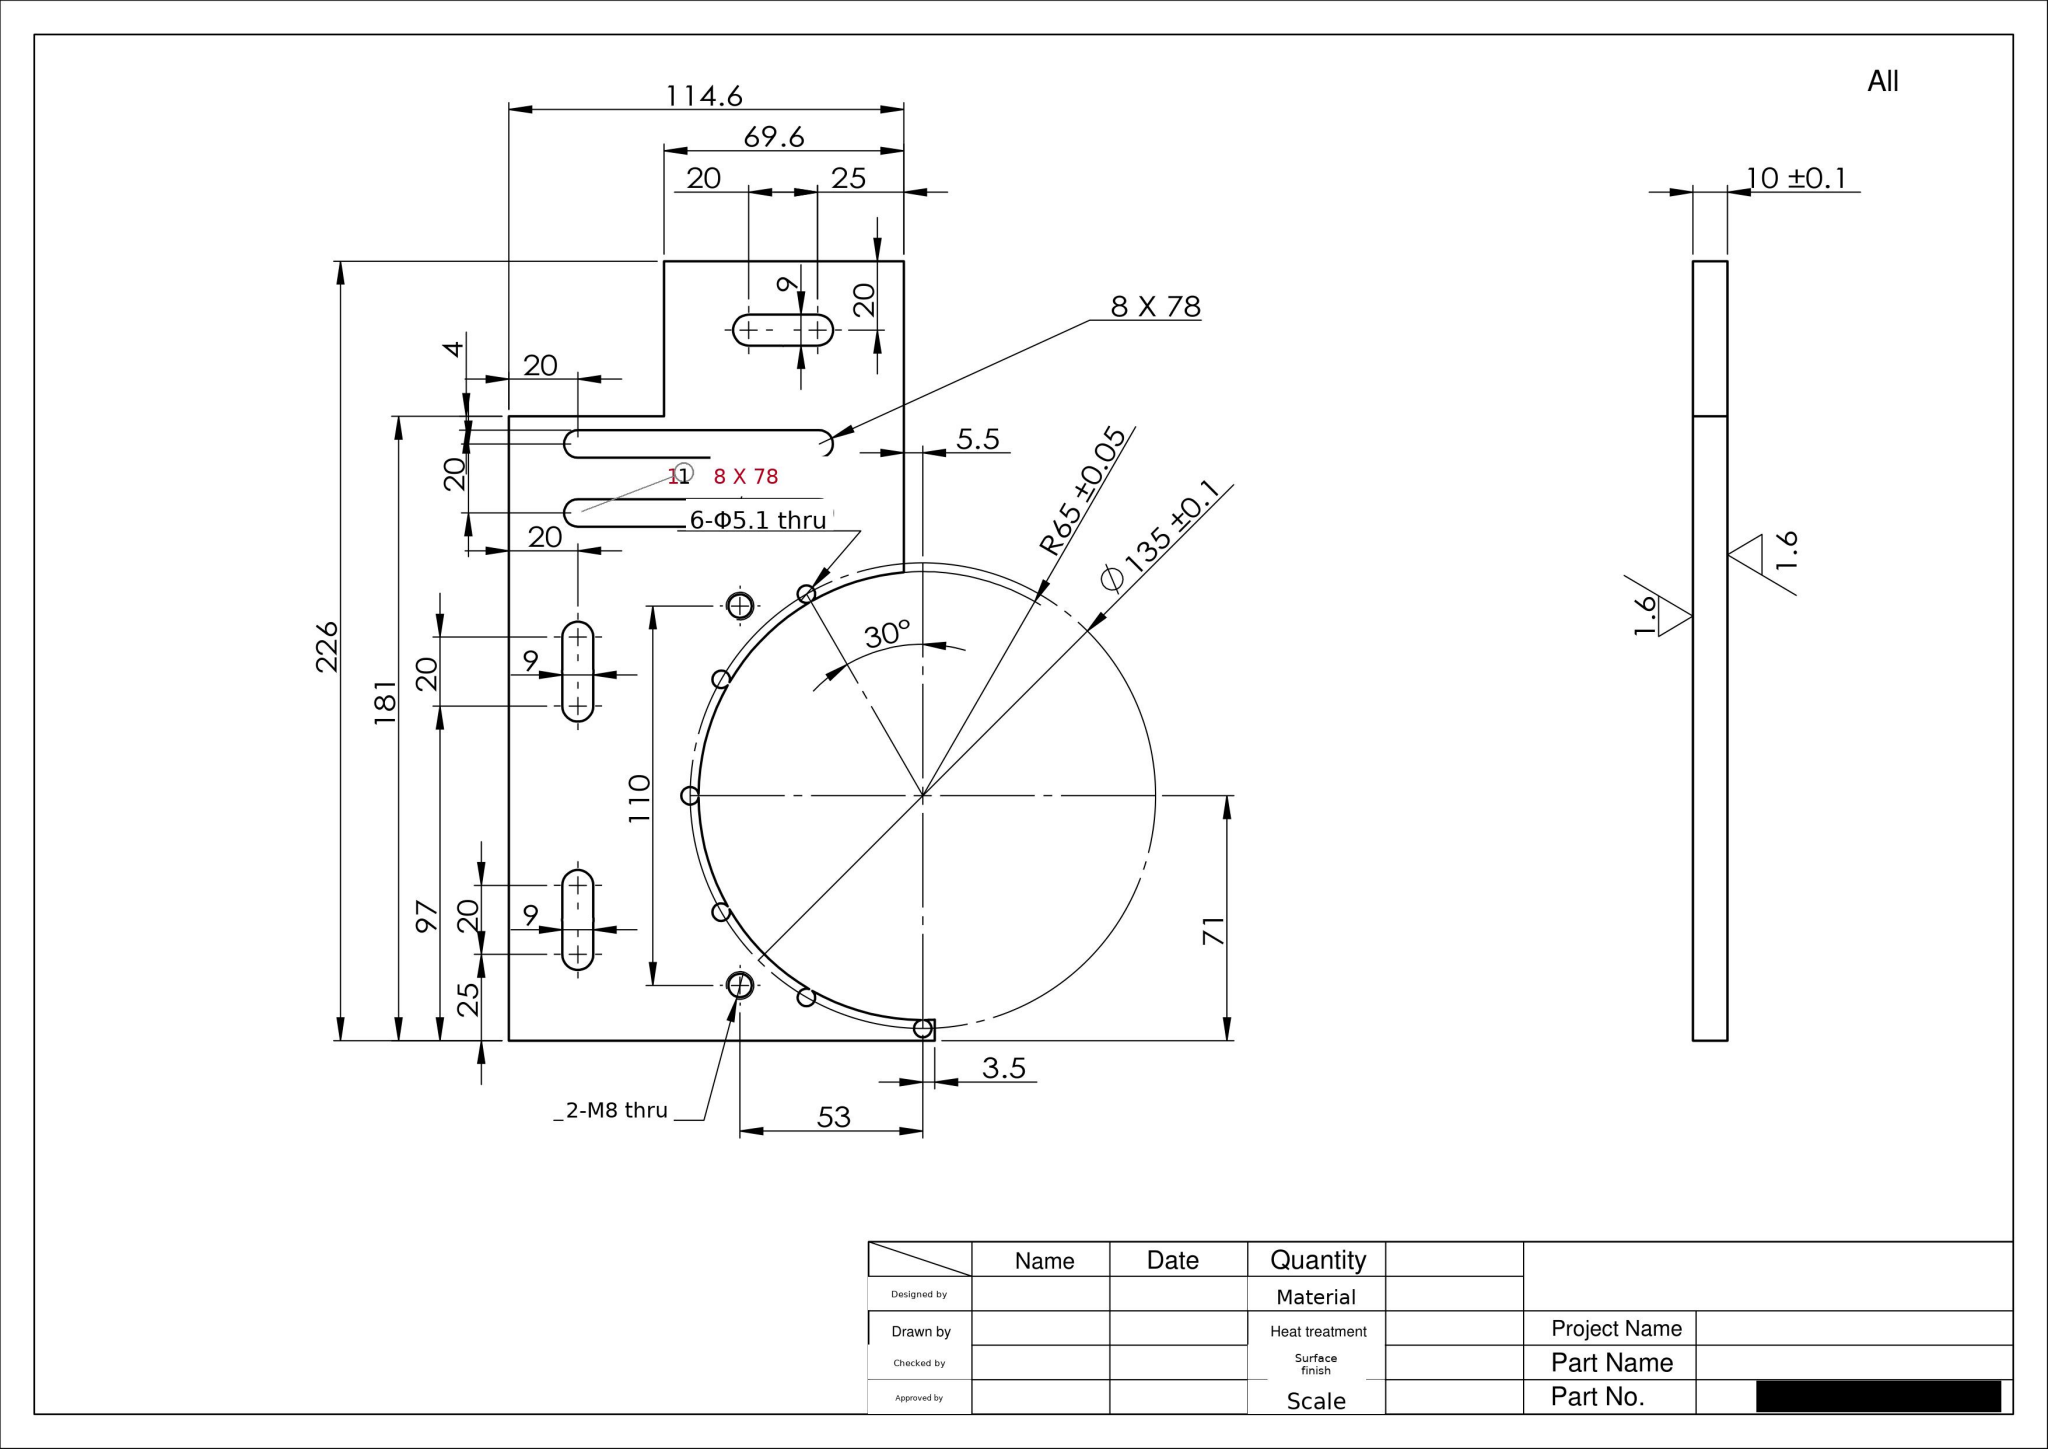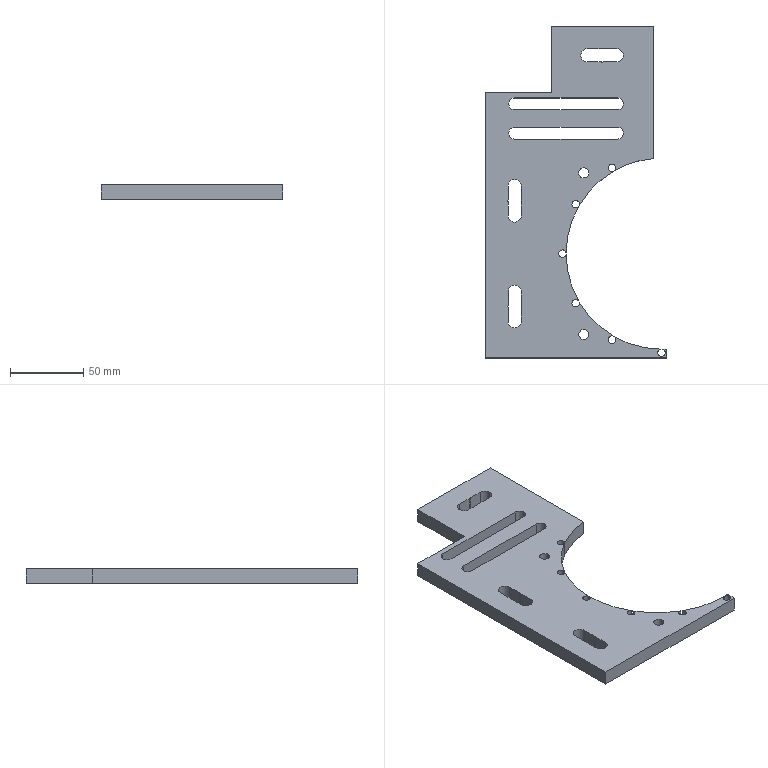Part | SolidWorks | mm | 1 solid | 74 faces | box 123.55 x 226 x 10 mm | volume 158487 mm3 | cylinder 49 | plane 25 | commonest cylinder face diameters 5.1 x17 9.1 x8 9 x7 130 x7 8 x6 6.8 x4